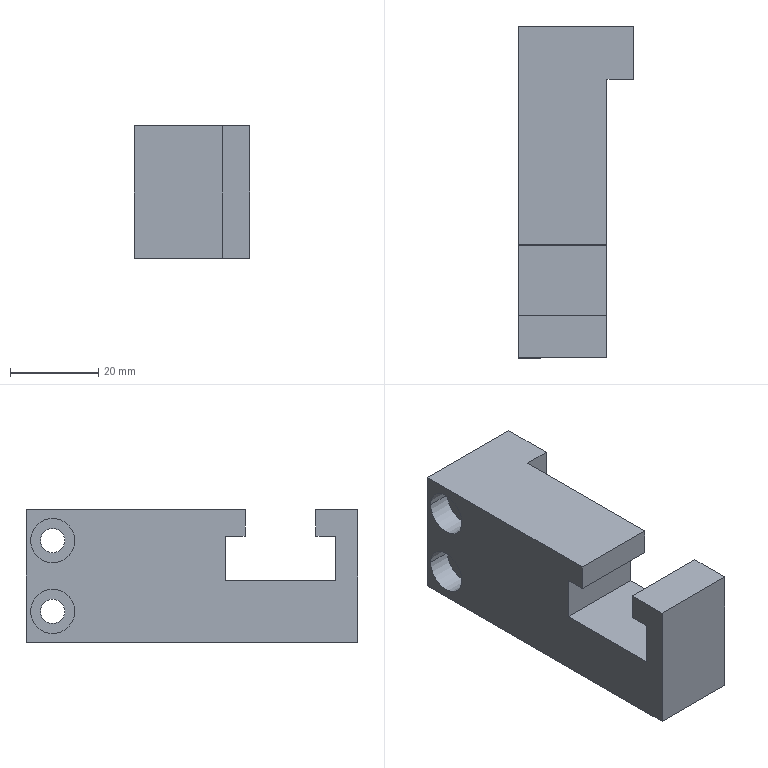Component | SolidWorks | 15-1 | 1 solid | 26 faces | box 26 x 75 x 30 mm | volume 38413 mm3 | plane 18 | cylinder 8 | commonest cylinder face diameters 10 x4 5.5 x4
build123d program:
from build123d import *

# Parameters (mm, degrees)
SKETCH1_W                                       = 30
SKETCH1_H                                       = 75
EXTRUDE1_DEPTH                                  = 10
CUT_EXTRUDE1_DEPTH                              = 46.069
SKETCH3_W                                       = 30
SKETCH3_H                                       = 12
EXTRUDE2_DEPTH                                  = 6
M5_HEX_SOCKET_HEAD_CAP_SCREW_CBORE1_D           = 5.5
M5_HEX_SOCKET_HEAD_CAP_SCREW_CBORE1_CBORE_D     = 10
M5_HEX_SOCKET_HEAD_CAP_SCREW_CBORE1_CBORE_DEPTH = 5.4


with BuildPart() as part:
    # Sketch1 → Extrude1 (new, symmetric)
    with BuildSketch(Plane(origin=(0, 0, 0), x_dir=(1, 0, 0), z_dir=(0, 1, 0))):
        Rectangle(SKETCH1_W, SKETCH1_H)
    extrude(amount=EXTRUDE1_DEPTH, both=True)

    # Sketch2 → Cut-Extrude1 (cut, through all)
    with BuildSketch(Plane.XZ.offset(10)):
        Polygon((15, 28), (9, 28), (9, 32.5), (-1, 32.5), (-1, 7.5), (9, 7.5), (9, 12), (15, 12), align=None)
    extrude(amount=-CUT_EXTRUDE1_DEPTH, mode=Mode.SUBTRACT)

    # Sketch3 → Extrude2 (add)
    with BuildSketch(Plane(origin=(0, -10, 0), x_dir=(1, 0, 0), z_dir=(0, 1, 0))):
        with Locations((0, 31.5)):
            Rectangle(SKETCH3_W, SKETCH3_H)
    extrude(amount=-EXTRUDE2_DEPTH)

    # M5 Hex Socket Head Cap Screw CBORE1 (through all)
    with Locations(Plane(origin=(0, 10, 0), x_dir=(1, 0, 0), z_dir=(0, 1, 0))):
        with Locations((8, 31.5), (-8, 31.5)):
            CounterBoreHole(M5_HEX_SOCKET_HEAD_CAP_SCREW_CBORE1_D / 2, M5_HEX_SOCKET_HEAD_CAP_SCREW_CBORE1_CBORE_D / 2, M5_HEX_SOCKET_HEAD_CAP_SCREW_CBORE1_CBORE_DEPTH)


solid = part.part

# Placed as in the assembly
solid = solid.moved(Location((-103, -9.5, 101.8), (90, 0, 90)))
STEP:
#1=COLOUR_RGB('',0.7922,0.8196,0.9333);
#2=FILL_AREA_STYLE_COLOUR('',#1);
#3=FILL_AREA_STYLE('',(#2));
#4=SURFACE_STYLE_FILL_AREA(#3);
#5=SURFACE_SIDE_STYLE('',(#4));
#6=SURFACE_STYLE_USAGE(.BOTH.,#5);
#7=PRESENTATION_STYLE_ASSIGNMENT((#6));
#8=CARTESIAN_POINT('',(-4.236,1.063,4.323));
#9=VERTEX_POINT('',#8);
#10=CARTESIAN_POINT('',(-4.236,0.6693,4.323));
#11=VERTEX_POINT('',#10);
#12=CARTESIAN_POINT('',(-4.236,0.8661,4.323));
#13=DIRECTION('',(-1.,-0.,0.));
#14=DIRECTION('',(0.,-1.,0.));
#15=AXIS2_PLACEMENT_3D('',#12,#13,#14);
#16=CIRCLE('',#15,0.1969);
#17=EDGE_CURVE('',#9,#11,#16,.T.);
#18=ORIENTED_EDGE('',*,*,#17,.F.);
#19=CARTESIAN_POINT('',(-4.449,1.063,4.323));
#20=VERTEX_POINT('',#19);
#21=CARTESIAN_POINT('',(-4.449,1.063,4.323));
#22=DIRECTION('',(-1.,-0.,0.));
#23=VECTOR('',#22,39.37);
#24=LINE('',#21,#23);
#25=EDGE_CURVE('',#9,#20,#24,.T.);
#26=ORIENTED_EDGE('',*,*,#25,.T.);
#27=CARTESIAN_POINT('',(-4.449,0.6693,4.323));
#28=VERTEX_POINT('',#27);
#29=CARTESIAN_POINT('',(-4.449,0.8661,4.323));
#30=DIRECTION('',(-1.,-0.,0.));
#31=DIRECTION('',(0.,-1.,0.));
#32=AXIS2_PLACEMENT_3D('',#29,#30,#31);
#33=CIRCLE('',#32,0.1969);
#34=EDGE_CURVE('',#20,#28,#33,.T.);
#35=ORIENTED_EDGE('',*,*,#34,.T.);
#36=CARTESIAN_POINT('',(-4.449,0.6693,4.323));
#37=DIRECTION('',(-1.,-0.,0.));
#38=VECTOR('',#37,39.37);
#39=LINE('',#36,#38);
#40=EDGE_CURVE('',#11,#28,#39,.T.);
#41=ORIENTED_EDGE('',*,*,#40,.F.);
#42=EDGE_LOOP('',(#18,#26,#35,#41));
#43=FACE_OUTER_BOUND('',#42,.T.);
#44=CARTESIAN_POINT('',(-4.449,0.8661,4.323));
#45=DIRECTION('',(-1.,-0.,0.));
#46=DIRECTION('',(0.,-1.,0.));
#47=AXIS2_PLACEMENT_3D('',#44,#45,#46);
#48=CYLINDRICAL_SURFACE('',#47,0.1969);
#49=ADVANCED_FACE('',(#43),#48,.F.);
#50=CARTESIAN_POINT('',(-3.425,0.9744,4.323));
#51=VERTEX_POINT('',#50);
#52=CARTESIAN_POINT('',(-3.425,0.7579,4.323));
#53=VERTEX_POINT('',#52);
#54=CARTESIAN_POINT('',(-3.425,0.8661,4.323));
#55=DIRECTION('',(-1.,-0.,0.));
#56=DIRECTION('',(0.,-1.,0.));
#57=AXIS2_PLACEMENT_3D('',#54,#55,#56);
#58=CIRCLE('',#57,0.1083);
#59=EDGE_CURVE('',#51,#53,#58,.T.);
#60=ORIENTED_EDGE('',*,*,#59,.F.);
#61=CARTESIAN_POINT('',(-4.236,0.9744,4.323));
#62=VERTEX_POINT('',#61);
#63=CARTESIAN_POINT('',(-4.449,0.9744,4.323));
#64=DIRECTION('',(-1.,-0.,0.));
#65=VECTOR('',#64,39.37);
#66=LINE('',#63,#65);
#67=EDGE_CURVE('',#51,#62,#66,.T.);
#68=ORIENTED_EDGE('',*,*,#67,.T.);
#69=CARTESIAN_POINT('',(-4.236,0.7579,4.323));
#70=VERTEX_POINT('',#69);
#71=CARTESIAN_POINT('',(-4.236,0.8661,4.323));
#72=DIRECTION('',(-1.,-0.,0.));
#73=DIRECTION('',(0.,-1.,0.));
#74=AXIS2_PLACEMENT_3D('',#71,#72,#73);
#75=CIRCLE('',#74,0.1083);
#76=EDGE_CURVE('',#62,#70,#75,.T.);
#77=ORIENTED_EDGE('',*,*,#76,.T.);
#78=CARTESIAN_POINT('',(-4.449,0.7579,4.323));
#79=DIRECTION('',(-1.,-0.,0.));
#80=VECTOR('',#79,39.37);
#81=LINE('',#78,#80);
#82=EDGE_CURVE('',#53,#70,#81,.T.);
#83=ORIENTED_EDGE('',*,*,#82,.F.);
#84=EDGE_LOOP('',(#60,#68,#77,#83));
#85=FACE_OUTER_BOUND('',#84,.T.);
#86=CARTESIAN_POINT('',(-4.449,0.8661,4.323));
#87=DIRECTION('',(-1.,-0.,0.));
#88=DIRECTION('',(0.,-1.,0.));
#89=AXIS2_PLACEMENT_3D('',#86,#87,#88);
#90=CYLINDRICAL_SURFACE('',#89,0.1083);
#91=ADVANCED_FACE('',(#85),#90,.F.);
#92=CARTESIAN_POINT('',(-4.236,1.063,3.693));
#93=VERTEX_POINT('',#92);
#94=CARTESIAN_POINT('',(-4.236,0.6693,3.693));
#95=VERTEX_POINT('',#94);
#96=CARTESIAN_POINT('',(-4.236,0.8661,3.693));
#97=DIRECTION('',(-1.,-0.,0.));
#98=DIRECTION('',(0.,-1.,0.));
#99=AXIS2_PLACEMENT_3D('',#96,#97,#98);
#100=CIRCLE('',#99,0.1969);
#101=EDGE_CURVE('',#93,#95,#100,.T.);
#102=ORIENTED_EDGE('',*,*,#101,.F.);
#103=CARTESIAN_POINT('',(-4.449,1.063,3.693));
#104=VERTEX_POINT('',#103);
#105=CARTESIAN_POINT('',(-4.449,1.063,3.693));
#106=DIRECTION('',(-1.,-0.,0.));
#107=VECTOR('',#106,39.37);
#108=LINE('',#105,#107);
#109=EDGE_CURVE('',#93,#104,#108,.T.);
#110=ORIENTED_EDGE('',*,*,#109,.T.);
#111=CARTESIAN_POINT('',(-4.449,0.6693,3.693));
#112=VERTEX_POINT('',#111);
#113=CARTESIAN_POINT('',(-4.449,0.8661,3.693));
#114=DIRECTION('',(-1.,-0.,0.));
#115=DIRECTION('',(0.,-1.,0.));
#116=AXIS2_PLACEMENT_3D('',#113,#114,#115);
#117=CIRCLE('',#116,0.1969);
#118=EDGE_CURVE('',#104,#112,#117,.T.);
#119=ORIENTED_EDGE('',*,*,#118,.T.);
#120=CARTESIAN_POINT('',(-4.449,0.6693,3.693));
#121=DIRECTION('',(-1.,-0.,0.));
#122=VECTOR('',#121,39.37);
#123=LINE('',#120,#122);
#124=EDGE_CURVE('',#95,#112,#123,.T.);
#125=ORIENTED_EDGE('',*,*,#124,.F.);
#126=EDGE_LOOP('',(#102,#110,#119,#125));
#127=FACE_OUTER_BOUND('',#126,.T.);
#128=CARTESIAN_POINT('',(-4.449,0.8661,3.693));
#129=DIRECTION('',(-1.,-0.,0.));
#130=DIRECTION('',(0.,-1.,0.));
#131=AXIS2_PLACEMENT_3D('',#128,#129,#130);
#132=CYLINDRICAL_SURFACE('',#131,0.1969);
#133=ADVANCED_FACE('',(#127),#132,.F.);
#134=CARTESIAN_POINT('',(-3.425,0.9744,3.693));
#135=VERTEX_POINT('',#134);
#136=CARTESIAN_POINT('',(-3.425,0.7579,3.693));
#137=VERTEX_POINT('',#136);
#138=CARTESIAN_POINT('',(-3.425,0.8661,3.693));
#139=DIRECTION('',(-1.,-0.,0.));
#140=DIRECTION('',(0.,-1.,0.));
#141=AXIS2_PLACEMENT_3D('',#138,#139,#140);
#142=CIRCLE('',#141,0.1083);
#143=EDGE_CURVE('',#135,#137,#142,.T.);
#144=ORIENTED_EDGE('',*,*,#143,.F.);
#145=CARTESIAN_POINT('',(-4.236,0.9744,3.693));
#146=VERTEX_POINT('',#145);
#147=CARTESIAN_POINT('',(-4.449,0.9744,3.693));
#148=DIRECTION('',(-1.,-0.,0.));
#149=VECTOR('',#148,39.37);
#150=LINE('',#147,#149);
#151=EDGE_CURVE('',#135,#146,#150,.T.);
#152=ORIENTED_EDGE('',*,*,#151,.T.);
#153=CARTESIAN_POINT('',(-4.236,0.7579,3.693));
#154=VERTEX_POINT('',#153);
#155=CARTESIAN_POINT('',(-4.236,0.8661,3.693));
#156=DIRECTION('',(-1.,-0.,0.));
#157=DIRECTION('',(0.,-1.,0.));
#158=AXIS2_PLACEMENT_3D('',#155,#156,#157);
#159=CIRCLE('',#158,0.1083);
#160=EDGE_CURVE('',#146,#154,#159,.T.);
#161=ORIENTED_EDGE('',*,*,#160,.T.);
#162=CARTESIAN_POINT('',(-4.449,0.7579,3.693));
#163=DIRECTION('',(-1.,-0.,0.));
#164=VECTOR('',#163,39.37);
#165=LINE('',#162,#164);
#166=EDGE_CURVE('',#137,#154,#165,.T.);
#167=ORIENTED_EDGE('',*,*,#166,.F.);
#168=EDGE_LOOP('',(#144,#152,#161,#167));
#169=FACE_OUTER_BOUND('',#168,.T.);
#170=CARTESIAN_POINT('',(-4.449,0.8661,3.693));
#171=DIRECTION('',(-1.,-0.,0.));
#172=DIRECTION('',(0.,-1.,0.));
#173=AXIS2_PLACEMENT_3D('',#170,#171,#172);
#174=CYLINDRICAL_SURFACE('',#173,0.1083);
#175=ADVANCED_FACE('',(#169),#174,.F.);
#176=CARTESIAN_POINT('',(-4.449,-0.8465,4.598));
#177=VERTEX_POINT('',#176);
#178=CARTESIAN_POINT('',(-4.449,1.102,4.598));
#179=VERTEX_POINT('',#178);
#180=CARTESIAN_POINT('',(-4.449,1.102,4.598));
#181=DIRECTION('',(-0.,1.,-0.));
#182=VECTOR('',#181,39.37);
#183=LINE('',#180,#182);
#184=EDGE_CURVE('',#177,#179,#183,.T.);
#185=ORIENTED_EDGE('',*,*,#184,.F.);
#186=CARTESIAN_POINT('',(-3.661,-0.8465,4.598));
#187=VERTEX_POINT('',#186);
#188=CARTESIAN_POINT('',(-4.449,-0.8465,4.598));
#189=DIRECTION('',(1.,0.,-0.));
#190=VECTOR('',#189,39.37);
#191=LINE('',#188,#190);
#192=EDGE_CURVE('',#177,#187,#191,.T.);
#193=ORIENTED_EDGE('',*,*,#192,.T.);
#194=CARTESIAN_POINT('',(-3.661,0.6299,4.598));
#195=VERTEX_POINT('',#194);
#196=CARTESIAN_POINT('',(-3.661,1.102,4.598));
#197=DIRECTION('',(-0.,1.,-0.));
#198=VECTOR('',#197,39.37);
#199=LINE('',#196,#198);
#200=EDGE_CURVE('',#187,#195,#199,.T.);
#201=ORIENTED_EDGE('',*,*,#200,.T.);
#202=CARTESIAN_POINT('',(-3.425,0.6299,4.598));
#203=VERTEX_POINT('',#202);
#204=CARTESIAN_POINT('',(-3.425,0.6299,4.598));
#205=DIRECTION('',(-1.,-0.,0.));
#206=VECTOR('',#205,39.37);
#207=LINE('',#204,#206);
#208=EDGE_CURVE('',#203,#195,#207,.T.);
#209=ORIENTED_EDGE('',*,*,#208,.F.);
#210=CARTESIAN_POINT('',(-3.425,1.102,4.598));
#211=VERTEX_POINT('',#210);
#212=CARTESIAN_POINT('',(-3.425,1.102,4.598));
#213=DIRECTION('',(-0.,1.,-0.));
#214=VECTOR('',#213,39.37);
#215=LINE('',#212,#214);
#216=EDGE_CURVE('',#203,#211,#215,.T.);
#217=ORIENTED_EDGE('',*,*,#216,.T.);
#218=CARTESIAN_POINT('',(-4.449,1.102,4.598));
#219=DIRECTION('',(1.,0.,-0.));
#220=VECTOR('',#219,39.37);
#221=LINE('',#218,#220);
#222=EDGE_CURVE('',#179,#211,#221,.T.);
#223=ORIENTED_EDGE('',*,*,#222,.F.);
#224=EDGE_LOOP('',(#185,#193,#201,#209,#217,#223));
#225=FACE_OUTER_BOUND('',#224,.T.);
#226=CARTESIAN_POINT('',(-4.449,1.102,4.598));
#227=DIRECTION('',(-0.,-0.,-1.));
#228=DIRECTION('',(0.,-1.,0.));
#229=AXIS2_PLACEMENT_3D('',#226,#227,#228);
#230=PLANE('',#229);
#231=ADVANCED_FACE('',(#225),#230,.F.);
#232=CARTESIAN_POINT('',(-4.449,1.102,3.417));
#233=VERTEX_POINT('',#232);
#234=CARTESIAN_POINT('',(-3.425,1.102,3.417));
#235=VERTEX_POINT('',#234);
#236=CARTESIAN_POINT('',(-4.449,1.102,3.417));
#237=DIRECTION('',(1.,0.,-0.));
#238=VECTOR('',#237,39.37);
#239=LINE('',#236,#238);
#240=EDGE_CURVE('',#233,#235,#239,.T.);
#241=ORIENTED_EDGE('',*,*,#240,.T.);
#242=CARTESIAN_POINT('',(-3.425,0.6299,3.417));
#243=VERTEX_POINT('',#242);
#244=CARTESIAN_POINT('',(-3.425,1.102,3.417));
#245=DIRECTION('',(0.,-1.,0.));
#246=VECTOR('',#245,39.37);
#247=LINE('',#244,#246);
#248=EDGE_CURVE('',#235,#243,#247,.T.);
#249=ORIENTED_EDGE('',*,*,#248,.T.);
#250=CARTESIAN_POINT('',(-3.661,0.6299,3.417));
#251=VERTEX_POINT('',#250);
#252=CARTESIAN_POINT('',(-3.425,0.6299,3.417));
#253=DIRECTION('',(-1.,-0.,0.));
#254=VECTOR('',#253,39.37);
#255=LINE('',#252,#254);
#256=EDGE_CURVE('',#243,#251,#255,.T.);
#257=ORIENTED_EDGE('',*,*,#256,.T.);
#258=CARTESIAN_POINT('',(-3.661,-1.85,3.417));
#259=VERTEX_POINT('',#258);
#260=CARTESIAN_POINT('',(-3.661,1.102,3.417));
#261=DIRECTION('',(0.,-1.,0.));
#262=VECTOR('',#261,39.37);
#263=LINE('',#260,#262);
#264=EDGE_CURVE('',#251,#259,#263,.T.);
#265=ORIENTED_EDGE('',*,*,#264,.T.);
#266=CARTESIAN_POINT('',(-4.449,-1.85,3.417));
#267=VERTEX_POINT('',#266);
#268=CARTESIAN_POINT('',(-4.449,-1.85,3.417));
#269=DIRECTION('',(1.,0.,-0.));
#270=VECTOR('',#269,39.37);
#271=LINE('',#268,#270);
#272=EDGE_CURVE('',#267,#259,#271,.T.);
#273=ORIENTED_EDGE('',*,*,#272,.F.);
#274=CARTESIAN_POINT('',(-4.449,1.102,3.417));
#275=DIRECTION('',(0.,-1.,0.));
#276=VECTOR('',#275,39.37);
#277=LINE('',#274,#276);
#278=EDGE_CURVE('',#233,#267,#277,.T.);
#279=ORIENTED_EDGE('',*,*,#278,.F.);
#280=EDGE_LOOP('',(#241,#249,#257,#265,#273,#279));
#281=FACE_OUTER_BOUND('',#280,.T.);
#282=CARTESIAN_POINT('',(-4.449,1.102,3.417));
#283=DIRECTION('',(0.,0.,1.));
#284=DIRECTION('',(-0.,1.,-0.));
#285=AXIS2_PLACEMENT_3D('',#282,#283,#284);
#286=PLANE('',#285);
#287=ADVANCED_FACE('',(#281),#286,.F.);
#288=CARTESIAN_POINT('',(-3.661,-1.85,4.598));
#289=VERTEX_POINT('',#288);
#290=CARTESIAN_POINT('',(-3.661,-1.85,3.417));
#291=DIRECTION('',(0.,0.,1.));
#292=VECTOR('',#291,39.37);
#293=LINE('',#290,#292);
#294=EDGE_CURVE('',#259,#289,#293,.T.);
#295=ORIENTED_EDGE('',*,*,#294,.T.);
#296=CARTESIAN_POINT('',(-4.449,-1.85,4.598));
#297=VERTEX_POINT('',#296);
#298=CARTESIAN_POINT('',(-4.449,-1.85,4.598));
#299=DIRECTION('',(1.,0.,-0.));
#300=VECTOR('',#299,39.37);
#301=LINE('',#298,#300);
#302=EDGE_CURVE('',#297,#289,#301,.T.);
#303=ORIENTED_EDGE('',*,*,#302,.F.);
#304=CARTESIAN_POINT('',(-4.449,-1.85,3.417));
#305=DIRECTION('',(0.,0.,1.));
#306=VECTOR('',#305,39.37);
#307=LINE('',#304,#306);
#308=EDGE_CURVE('',#267,#297,#307,.T.);
#309=ORIENTED_EDGE('',*,*,#308,.F.);
#310=ORIENTED_EDGE('',*,*,#272,.T.);
#311=EDGE_LOOP('',(#295,#303,#309,#310));
#312=FACE_OUTER_BOUND('',#311,.T.);
#313=CARTESIAN_POINT('',(-4.449,-1.85,3.417));
#314=DIRECTION('',(-0.,1.,-0.));
#315=DIRECTION('',(-0.,-0.,-1.));
#316=AXIS2_PLACEMENT_3D('',#313,#314,#315);
#317=PLANE('',#316);
#318=ADVANCED_FACE('',(#312),#317,.F.);
#319=CARTESIAN_POINT('',(-3.661,-1.476,4.598));
#320=VERTEX_POINT('',#319);
#321=CARTESIAN_POINT('',(-3.661,1.102,4.598));
#322=DIRECTION('',(-0.,1.,-0.));
#323=VECTOR('',#322,39.37);
#324=LINE('',#321,#323);
#325=EDGE_CURVE('',#289,#320,#324,.T.);
#326=ORIENTED_EDGE('',*,*,#325,.T.);
#327=CARTESIAN_POINT('',(-4.449,-1.476,4.598));
#328=VERTEX_POINT('',#327);
#329=CARTESIAN_POINT('',(-4.449,-1.476,4.598));
#330=DIRECTION('',(1.,0.,-0.));
#331=VECTOR('',#330,39.37);
#332=LINE('',#329,#331);
#333=EDGE_CURVE('',#328,#320,#332,.T.);
#334=ORIENTED_EDGE('',*,*,#333,.F.);
#335=CARTESIAN_POINT('',(-4.449,1.102,4.598));
#336=DIRECTION('',(-0.,1.,-0.));
#337=VECTOR('',#336,39.37);
#338=LINE('',#335,#337);
#339=EDGE_CURVE('',#297,#328,#338,.T.);
#340=ORIENTED_EDGE('',*,*,#339,.F.);
#341=ORIENTED_EDGE('',*,*,#302,.T.);
#342=EDGE_LOOP('',(#326,#334,#340,#341));
#343=FACE_OUTER_BOUND('',#342,.T.);
#344=CARTESIAN_POINT('',(-4.449,1.102,4.598));
#345=DIRECTION('',(-0.,-0.,-1.));
#346=DIRECTION('',(0.,-1.,0.));
#347=AXIS2_PLACEMENT_3D('',#344,#345,#346);
#348=PLANE('',#347);
#349=ADVANCED_FACE('',(#343),#348,.F.);
#350=ORIENTED_EDGE('',*,*,#222,.T.);
#351=CARTESIAN_POINT('',(-3.425,1.102,3.417));
#352=DIRECTION('',(-0.,-0.,-1.));
#353=VECTOR('',#352,39.37);
#354=LINE('',#351,#353);
#355=EDGE_CURVE('',#211,#235,#354,.T.);
#356=ORIENTED_EDGE('',*,*,#355,.T.);
#357=ORIENTED_EDGE('',*,*,#240,.F.);
#358=CARTESIAN_POINT('',(-4.449,1.102,3.417));
#359=DIRECTION('',(-0.,-0.,-1.));
#360=VECTOR('',#359,39.37);
#361=LINE('',#358,#360);
#362=EDGE_CURVE('',#179,#233,#361,.T.);
#363=ORIENTED_EDGE('',*,*,#362,.F.);
#364=EDGE_LOOP('',(#350,#356,#357,#363));
#365=FACE_OUTER_BOUND('',#364,.T.);
#366=CARTESIAN_POINT('',(-4.449,1.102,3.417));
#367=DIRECTION('',(0.,-1.,0.));
#368=DIRECTION('',(0.,0.,1.));
#369=AXIS2_PLACEMENT_3D('',#366,#367,#368);
#370=PLANE('',#369);
#371=ADVANCED_FACE('',(#365),#370,.F.);
#372=CARTESIAN_POINT('',(-4.449,0.8661,4.323));
#373=DIRECTION('',(-1.,-0.,0.));
#374=DIRECTION('',(0.,-1.,0.));
#375=AXIS2_PLACEMENT_3D('',#372,#373,#374);
#376=CIRCLE('',#375,0.1969);
#377=EDGE_CURVE('',#28,#20,#376,.T.);
#378=ORIENTED_EDGE('',*,*,#377,.F.);
#379=ORIENTED_EDGE('',*,*,#34,.F.);
#380=EDGE_LOOP('',(#378,#379));
#381=FACE_BOUND('',#380,.T.);
#382=CARTESIAN_POINT('',(-4.449,0.8661,3.693));
#383=DIRECTION('',(-1.,-0.,0.));
#384=DIRECTION('',(0.,-1.,0.));
#385=AXIS2_PLACEMENT_3D('',#382,#383,#384);
#386=CIRCLE('',#385,0.1969);
#387=EDGE_CURVE('',#112,#104,#386,.T.);
#388=ORIENTED_EDGE('',*,*,#387,.F.);
#389=ORIENTED_EDGE('',*,*,#118,.F.);
#390=EDGE_LOOP('',(#388,#389));
#391=FACE_BOUND('',#390,.T.);
#392=CARTESIAN_POINT('',(-4.449,-0.8465,4.362));
#393=VERTEX_POINT('',#392);
#394=CARTESIAN_POINT('',(-4.449,-0.8465,4.362));
#395=DIRECTION('',(0.,0.,1.));
#396=VECTOR('',#395,39.37);
#397=LINE('',#394,#396);
#398=EDGE_CURVE('',#393,#177,#397,.T.);
#399=ORIENTED_EDGE('',*,*,#398,.T.);
#400=ORIENTED_EDGE('',*,*,#184,.T.);
#401=ORIENTED_EDGE('',*,*,#362,.T.);
#402=ORIENTED_EDGE('',*,*,#278,.T.);
#403=ORIENTED_EDGE('',*,*,#308,.T.);
#404=ORIENTED_EDGE('',*,*,#339,.T.);
#405=CARTESIAN_POINT('',(-4.449,-1.476,4.362));
#406=VERTEX_POINT('',#405);
#407=CARTESIAN_POINT('',(-4.449,-1.476,4.598));
#408=DIRECTION('',(-0.,-0.,-1.));
#409=VECTOR('',#408,39.37);
#410=LINE('',#407,#409);
#411=EDGE_CURVE('',#328,#406,#410,.T.);
#412=ORIENTED_EDGE('',*,*,#411,.T.);
#413=CARTESIAN_POINT('',(-4.449,-1.654,4.362));
#414=VERTEX_POINT('',#413);
#415=CARTESIAN_POINT('',(-4.449,-1.476,4.362));
#416=DIRECTION('',(0.,-1.,0.));
#417=VECTOR('',#416,39.37);
#418=LINE('',#415,#417);
#419=EDGE_CURVE('',#406,#414,#418,.T.);
#420=ORIENTED_EDGE('',*,*,#419,.T.);
#421=CARTESIAN_POINT('',(-4.449,-1.654,3.969));
#422=VERTEX_POINT('',#421);
#423=CARTESIAN_POINT('',(-4.449,-1.654,4.362));
#424=DIRECTION('',(-0.,-0.,-1.));
#425=VECTOR('',#424,39.37);
#426=LINE('',#423,#425);
#427=EDGE_CURVE('',#414,#422,#426,.T.);
#428=ORIENTED_EDGE('',*,*,#427,.T.);
#429=CARTESIAN_POINT('',(-4.449,-0.6693,3.969));
#430=VERTEX_POINT('',#429);
#431=CARTESIAN_POINT('',(-4.449,-1.654,3.969));
#432=DIRECTION('',(-0.,1.,-0.));
#433=VECTOR('',#432,39.37);
#434=LINE('',#431,#433);
#435=EDGE_CURVE('',#422,#430,#434,.T.);
#436=ORIENTED_EDGE('',*,*,#435,.T.);
#437=CARTESIAN_POINT('',(-4.449,-0.6693,4.362));
#438=VERTEX_POINT('',#437);
#439=CARTESIAN_POINT('',(-4.449,-0.6693,3.969));
#440=DIRECTION('',(0.,0.,1.));
#441=VECTOR('',#440,39.37);
#442=LINE('',#439,#441);
#443=EDGE_CURVE('',#430,#438,#442,.T.);
#444=ORIENTED_EDGE('',*,*,#443,.T.);
#445=CARTESIAN_POINT('',(-4.449,-0.6693,4.362));
#446=DIRECTION('',(0.,-1.,0.));
#447=VECTOR('',#446,39.37);
#448=LINE('',#445,#447);
#449=EDGE_CURVE('',#438,#393,#448,.T.);
#450=ORIENTED_EDGE('',*,*,#449,.T.);
#451=EDGE_LOOP('',(#399,#400,#401,#402,#403,#404,#412,#420,#428,#436,#444,#450));
#452=FACE_OUTER_BOUND('',#451,.T.);
#453=CARTESIAN_POINT('',(-4.449,-0.374,4.008));
#454=DIRECTION('',(-1.,-0.,0.));
#455=DIRECTION('',(0.,-1.,0.));
#456=AXIS2_PLACEMENT_3D('',#453,#454,#455);
#457=PLANE('',#456);
#458=ADVANCED_FACE('',(#381,#391,#452),#457,.T.);
#459=ORIENTED_EDGE('',*,*,#264,.F.);
#460=CARTESIAN_POINT('',(-3.661,0.6299,3.417));
#461=DIRECTION('',(0.,0.,1.));
#462=VECTOR('',#461,39.37);
#463=LINE('',#460,#462);
#464=EDGE_CURVE('',#251,#195,#463,.T.);
#465=ORIENTED_EDGE('',*,*,#464,.T.);
#466=ORIENTED_EDGE('',*,*,#200,.F.);
#467=CARTESIAN_POINT('',(-3.661,-0.8465,4.362));
#468=VERTEX_POINT('',#467);
#469=CARTESIAN_POINT('',(-3.661,-0.8465,4.362));
#470=DIRECTION('',(0.,0.,1.));
#471=VECTOR('',#470,39.37);
#472=LINE('',#469,#471);
#473=EDGE_CURVE('',#468,#187,#472,.T.);
#474=ORIENTED_EDGE('',*,*,#473,.F.);
#475=CARTESIAN_POINT('',(-3.661,-0.6693,4.362));
#476=VERTEX_POINT('',#475);
#477=CARTESIAN_POINT('',(-3.661,-0.6693,4.362));
#478=DIRECTION('',(0.,-1.,0.));
#479=VECTOR('',#478,39.37);
#480=LINE('',#477,#479);
#481=EDGE_CURVE('',#476,#468,#480,.T.);
#482=ORIENTED_EDGE('',*,*,#481,.F.);
#483=CARTESIAN_POINT('',(-3.661,-0.6693,3.969));
#484=VERTEX_POINT('',#483);
#485=CARTESIAN_POINT('',(-3.661,-0.6693,3.969));
#486=DIRECTION('',(0.,0.,1.));
#487=VECTOR('',#486,39.37);
#488=LINE('',#485,#487);
#489=EDGE_CURVE('',#484,#476,#488,.T.);
#490=ORIENTED_EDGE('',*,*,#489,.F.);
#491=CARTESIAN_POINT('',(-3.661,-1.654,3.969));
#492=VERTEX_POINT('',#491);
#493=CARTESIAN_POINT('',(-3.661,-1.654,3.969));
#494=DIRECTION('',(-0.,1.,-0.));
#495=VECTOR('',#494,39.37);
#496=LINE('',#493,#495);
#497=EDGE_CURVE('',#492,#484,#496,.T.);
#498=ORIENTED_EDGE('',*,*,#497,.F.);
#499=CARTESIAN_POINT('',(-3.661,-1.654,4.362));
#500=VERTEX_POINT('',#499);
#501=CARTESIAN_POINT('',(-3.661,-1.654,4.362));
#502=DIRECTION('',(-0.,-0.,-1.));
#503=VECTOR('',#502,39.37);
#504=LINE('',#501,#503);
#505=EDGE_CURVE('',#500,#492,#504,.T.);
#506=ORIENTED_EDGE('',*,*,#505,.F.);
#507=CARTESIAN_POINT('',(-3.661,-1.476,4.362));
#508=VERTEX_POINT('',#507);
#509=CARTESIAN_POINT('',(-3.661,-1.476,4.362));
#510=DIRECTION('',(0.,-1.,0.));
#511=VECTOR('',#510,39.37);
#512=LINE('',#509,#511);
#513=EDGE_CURVE('',#508,#500,#512,.T.);
#514=ORIENTED_EDGE('',*,*,#513,.F.);
#515=CARTESIAN_POINT('',(-3.661,-1.476,4.598));
#516=DIRECTION('',(-0.,-0.,-1.));
#517=VECTOR('',#516,39.37);
#518=LINE('',#515,#517);
#519=EDGE_CURVE('',#320,#508,#518,.T.);
#520=ORIENTED_EDGE('',*,*,#519,.F.);
#521=ORIENTED_EDGE('',*,*,#325,.F.);
#522=ORIENTED_EDGE('',*,*,#294,.F.);
#523=EDGE_LOOP('',(#459,#465,#466,#474,#482,#490,#498,#506,#514,#520,#521,#522));
#524=FACE_OUTER_BOUND('',#523,.T.);
#525=CARTESIAN_POINT('',(-3.661,-0.374,4.008));
#526=DIRECTION('',(-1.,-0.,0.));
#527=DIRECTION('',(0.,-1.,0.));
#528=AXIS2_PLACEMENT_3D('',#525,#526,#527);
#529=PLANE('',#528);
#530=ADVANCED_FACE('',(#524),#529,.F.);
#531=ORIENTED_EDGE('',*,*,#473,.T.);
#532=ORIENTED_EDGE('',*,*,#192,.F.);
#533=ORIENTED_EDGE('',*,*,#398,.F.);
#534=CARTESIAN_POINT('',(-4.449,-0.8465,4.362));
#535=DIRECTION('',(1.,0.,-0.));
#536=VECTOR('',#535,39.37);
#537=LINE('',#534,#536);
#538=EDGE_CURVE('',#393,#468,#537,.T.);
#539=ORIENTED_EDGE('',*,*,#538,.T.);
#540=EDGE_LOOP('',(#531,#532,#533,#539));
#541=FACE_OUTER_BOUND('',#540,.T.);
#542=CARTESIAN_POINT('',(-4.449,-0.8465,4.362));
#543=DIRECTION('',(-0.,1.,-0.));
#544=DIRECTION('',(-0.,-0.,-1.));
#545=AXIS2_PLACEMENT_3D('',#542,#543,#544);
#546=PLANE('',#545);
#547=ADVANCED_FACE('',(#541),#546,.F.);
#548=ORIENTED_EDGE('',*,*,#481,.T.);
#549=ORIENTED_EDGE('',*,*,#538,.F.);
#550=ORIENTED_EDGE('',*,*,#449,.F.);
#551=CARTESIAN_POINT('',(-4.449,-0.6693,4.362));
#552=DIRECTION('',(1.,0.,-0.));
#553=VECTOR('',#552,39.37);
#554=LINE('',#551,#553);
#555=EDGE_CURVE('',#438,#476,#554,.T.);
#556=ORIENTED_EDGE('',*,*,#555,.T.);
#557=EDGE_LOOP('',(#548,#549,#550,#556));
#558=FACE_OUTER_BOUND('',#557,.T.);
#559=CARTESIAN_POINT('',(-4.449,-0.6693,4.362));
#560=DIRECTION('',(0.,0.,1.));
#561=DIRECTION('',(-0.,1.,-0.));
#562=AXIS2_PLACEMENT_3D('',#559,#560,#561);
#563=PLANE('',#562);
#564=ADVANCED_FACE('',(#558),#563,.F.);
#565=ORIENTED_EDGE('',*,*,#489,.T.);
#566=ORIENTED_EDGE('',*,*,#555,.F.);
#567=ORIENTED_EDGE('',*,*,#443,.F.);
#568=CARTESIAN_POINT('',(-4.449,-0.6693,3.969));
#569=DIRECTION('',(1.,0.,-0.));
#570=VECTOR('',#569,39.37);
#571=LINE('',#568,#570);
#572=EDGE_CURVE('',#430,#484,#571,.T.);
#573=ORIENTED_EDGE('',*,*,#572,.T.);
#574=EDGE_LOOP('',(#565,#566,#567,#573));
#575=FACE_OUTER_BOUND('',#574,.T.);
#576=CARTESIAN_POINT('',(-4.449,-0.6693,3.969));
#577=DIRECTION('',(-0.,1.,-0.));
#578=DIRECTION('',(-0.,-0.,-1.));
#579=AXIS2_PLACEMENT_3D('',#576,#577,#578);
#580=PLANE('',#579);
#581=ADVANCED_FACE('',(#575),#580,.F.);
#582=ORIENTED_EDGE('',*,*,#497,.T.);
#583=ORIENTED_EDGE('',*,*,#572,.F.);
#584=ORIENTED_EDGE('',*,*,#435,.F.);
#585=CARTESIAN_POINT('',(-4.449,-1.654,3.969));
#586=DIRECTION('',(1.,0.,-0.));
#587=VECTOR('',#586,39.37);
#588=LINE('',#585,#587);
#589=EDGE_CURVE('',#422,#492,#588,.T.);
#590=ORIENTED_EDGE('',*,*,#589,.T.);
#591=EDGE_LOOP('',(#582,#583,#584,#590));
#592=FACE_OUTER_BOUND('',#591,.T.);
#593=CARTESIAN_POINT('',(-4.449,-1.654,3.969));
#594=DIRECTION('',(-0.,-0.,-1.));
#595=DIRECTION('',(0.,-1.,0.));
#596=AXIS2_PLACEMENT_3D('',#593,#594,#595);
#597=PLANE('',#596);
#598=ADVANCED_FACE('',(#592),#597,.F.);
#599=ORIENTED_EDGE('',*,*,#505,.T.);
#600=ORIENTED_EDGE('',*,*,#589,.F.);
#601=ORIENTED_EDGE('',*,*,#427,.F.);
#602=CARTESIAN_POINT('',(-4.449,-1.654,4.362));
#603=DIRECTION('',(1.,0.,-0.));
#604=VECTOR('',#603,39.37);
#605=LINE('',#602,#604);
#606=EDGE_CURVE('',#414,#500,#605,.T.);
#607=ORIENTED_EDGE('',*,*,#606,.T.);
#608=EDGE_LOOP('',(#599,#600,#601,#607));
#609=FACE_OUTER_BOUND('',#608,.T.);
#610=CARTESIAN_POINT('',(-4.449,-1.654,4.362));
#611=DIRECTION('',(0.,-1.,0.));
#612=DIRECTION('',(0.,0.,1.));
#613=AXIS2_PLACEMENT_3D('',#610,#611,#612);
#614=PLANE('',#613);
#615=ADVANCED_FACE('',(#609),#614,.F.);
#616=ORIENTED_EDGE('',*,*,#513,.T.);
#617=ORIENTED_EDGE('',*,*,#606,.F.);
#618=ORIENTED_EDGE('',*,*,#419,.F.);
#619=CARTESIAN_POINT('',(-4.449,-1.476,4.362));
#620=DIRECTION('',(1.,0.,-0.));
#621=VECTOR('',#620,39.37);
#622=LINE('',#619,#621);
#623=EDGE_CURVE('',#406,#508,#622,.T.);
#624=ORIENTED_EDGE('',*,*,#623,.T.);
#625=EDGE_LOOP('',(#616,#617,#618,#624));
#626=FACE_OUTER_BOUND('',#625,.T.);
#627=CARTESIAN_POINT('',(-4.449,-1.476,4.362));
#628=DIRECTION('',(0.,0.,1.));
#629=DIRECTION('',(-0.,1.,-0.));
#630=AXIS2_PLACEMENT_3D('',#627,#628,#629);
#631=PLANE('',#630);
#632=ADVANCED_FACE('',(#626),#631,.F.);
#633=ORIENTED_EDGE('',*,*,#519,.T.);
#634=ORIENTED_EDGE('',*,*,#623,.F.);
#635=ORIENTED_EDGE('',*,*,#411,.F.);
#636=ORIENTED_EDGE('',*,*,#333,.T.);
#637=EDGE_LOOP('',(#633,#634,#635,#636));
#638=FACE_OUTER_BOUND('',#637,.T.);
#639=CARTESIAN_POINT('',(-4.449,-1.476,4.598));
#640=DIRECTION('',(0.,-1.,0.));
#641=DIRECTION('',(0.,0.,1.));
#642=AXIS2_PLACEMENT_3D('',#639,#640,#641);
#643=PLANE('',#642);
#644=ADVANCED_FACE('',(#638),#643,.F.);
#645=ORIENTED_EDGE('',*,*,#464,.F.);
#646=ORIENTED_EDGE('',*,*,#256,.F.);
#647=CARTESIAN_POINT('',(-3.425,0.6299,3.417));
#648=DIRECTION('',(0.,0.,1.));
#649=VECTOR('',#648,39.37);
#650=LINE('',#647,#649);
#651=EDGE_CURVE('',#243,#203,#650,.T.);
#652=ORIENTED_EDGE('',*,*,#651,.T.);
#653=ORIENTED_EDGE('',*,*,#208,.T.);
#654=EDGE_LOOP('',(#645,#646,#652,#653));
#655=FACE_OUTER_BOUND('',#654,.T.);
#656=CARTESIAN_POINT('',(-3.425,0.6299,3.417));
#657=DIRECTION('',(0.,-1.,0.));
#658=DIRECTION('',(0.,0.,1.));
#659=AXIS2_PLACEMENT_3D('',#656,#657,#658);
#660=PLANE('',#659);
#661=ADVANCED_FACE('',(#655),#660,.T.);
#662=CARTESIAN_POINT('',(-3.425,0.8661,4.323));
#663=DIRECTION('',(-1.,-0.,0.));
#664=DIRECTION('',(0.,-1.,0.));
#665=AXIS2_PLACEMENT_3D('',#662,#663,#664);
#666=CIRCLE('',#665,0.1083);
#667=EDGE_CURVE('',#53,#51,#666,.T.);
#668=ORIENTED_EDGE('',*,*,#667,.T.);
#669=ORIENTED_EDGE('',*,*,#59,.T.);
#670=EDGE_LOOP('',(#668,#669));
#671=FACE_BOUND('',#670,.T.);
#672=CARTESIAN_POINT('',(-3.425,0.8661,3.693));
#673=DIRECTION('',(-1.,-0.,0.));
#674=DIRECTION('',(0.,-1.,0.));
#675=AXIS2_PLACEMENT_3D('',#672,#673,#674);
#676=CIRCLE('',#675,0.1083);
#677=EDGE_CURVE('',#137,#135,#676,.T.);
#678=ORIENTED_EDGE('',*,*,#677,.T.);
#679=ORIENTED_EDGE('',*,*,#143,.T.);
#680=EDGE_LOOP('',(#678,#679));
#681=FACE_BOUND('',#680,.T.);
#682=ORIENTED_EDGE('',*,*,#248,.F.);
#683=ORIENTED_EDGE('',*,*,#355,.F.);
#684=ORIENTED_EDGE('',*,*,#216,.F.);
#685=ORIENTED_EDGE('',*,*,#651,.F.);
#686=EDGE_LOOP('',(#682,#683,#684,#685));
#687=FACE_OUTER_BOUND('',#686,.T.);
#688=CARTESIAN_POINT('',(-3.425,-0.374,4.008));
#689=DIRECTION('',(-1.,-0.,0.));
#690=DIRECTION('',(0.,-1.,0.));
#691=AXIS2_PLACEMENT_3D('',#688,#689,#690);
#692=PLANE('',#691);
#693=ADVANCED_FACE('',(#671,#681,#687),#692,.F.);
#694=ORIENTED_EDGE('',*,*,#151,.F.);
#695=ORIENTED_EDGE('',*,*,#677,.F.);
#696=ORIENTED_EDGE('',*,*,#166,.T.);
#697=CARTESIAN_POINT('',(-4.236,0.8661,3.693));
#698=DIRECTION('',(-1.,-0.,0.));
#699=DIRECTION('',(0.,-1.,0.));
#700=AXIS2_PLACEMENT_3D('',#697,#698,#699);
#701=CIRCLE('',#700,0.1083);
#702=EDGE_CURVE('',#154,#146,#701,.T.);
#703=ORIENTED_EDGE('',*,*,#702,.T.);
#704=EDGE_LOOP('',(#694,#695,#696,#703));
#705=FACE_OUTER_BOUND('',#704,.T.);
#706=CARTESIAN_POINT('',(-4.449,0.8661,3.693));
#707=DIRECTION('',(-1.,-0.,0.));
#708=DIRECTION('',(0.,-1.,0.));
#709=AXIS2_PLACEMENT_3D('',#706,#707,#708);
#710=CYLINDRICAL_SURFACE('',#709,0.1083);
#711=ADVANCED_FACE('',(#705),#710,.F.);
#712=ORIENTED_EDGE('',*,*,#702,.F.);
#713=ORIENTED_EDGE('',*,*,#160,.F.);
#714=EDGE_LOOP('',(#712,#713));
#715=FACE_BOUND('',#714,.T.);
#716=CARTESIAN_POINT('',(-4.236,0.8661,3.693));
#717=DIRECTION('',(-1.,-0.,0.));
#718=DIRECTION('',(0.,-1.,0.));
#719=AXIS2_PLACEMENT_3D('',#716,#717,#718);
#720=CIRCLE('',#719,0.1969);
#721=EDGE_CURVE('',#95,#93,#720,.T.);
#722=ORIENTED_EDGE('',*,*,#721,.T.);
#723=ORIENTED_EDGE('',*,*,#101,.T.);
#724=EDGE_LOOP('',(#722,#723));
#725=FACE_OUTER_BOUND('',#724,.T.);
#726=CARTESIAN_POINT('',(-4.236,0.8661,3.801));
#727=DIRECTION('',(1.,0.,-0.));
#728=DIRECTION('',(-0.,1.,-0.));
#729=AXIS2_PLACEMENT_3D('',#726,#727,#728);
#730=PLANE('',#729);
#731=ADVANCED_FACE('',(#715,#725),#730,.F.);
#732=ORIENTED_EDGE('',*,*,#109,.F.);
#733=ORIENTED_EDGE('',*,*,#721,.F.);
#734=ORIENTED_EDGE('',*,*,#124,.T.);
#735=ORIENTED_EDGE('',*,*,#387,.T.);
#736=EDGE_LOOP('',(#732,#733,#734,#735));
#737=FACE_OUTER_BOUND('',#736,.T.);
#738=CARTESIAN_POINT('',(-4.449,0.8661,3.693));
#739=DIRECTION('',(-1.,-0.,0.));
#740=DIRECTION('',(0.,-1.,0.));
#741=AXIS2_PLACEMENT_3D('',#738,#739,#740);
#742=CYLINDRICAL_SURFACE('',#741,0.1969);
#743=ADVANCED_FACE('',(#737),#742,.F.);
#744=ORIENTED_EDGE('',*,*,#67,.F.);
#745=ORIENTED_EDGE('',*,*,#667,.F.);
#746=ORIENTED_EDGE('',*,*,#82,.T.);
#747=CARTESIAN_POINT('',(-4.236,0.8661,4.323));
#748=DIRECTION('',(-1.,-0.,0.));
#749=DIRECTION('',(0.,-1.,0.));
#750=AXIS2_PLACEMENT_3D('',#747,#748,#749);
#751=CIRCLE('',#750,0.1083);
#752=EDGE_CURVE('',#70,#62,#751,.T.);
#753=ORIENTED_EDGE('',*,*,#752,.T.);
#754=EDGE_LOOP('',(#744,#745,#746,#753));
#755=FACE_OUTER_BOUND('',#754,.T.);
#756=CARTESIAN_POINT('',(-4.449,0.8661,4.323));
#757=DIRECTION('',(-1.,-0.,0.));
#758=DIRECTION('',(0.,-1.,0.));
#759=AXIS2_PLACEMENT_3D('',#756,#757,#758);
#760=CYLINDRICAL_SURFACE('',#759,0.1083);
#761=ADVANCED_FACE('',(#755),#760,.F.);
#762=ORIENTED_EDGE('',*,*,#752,.F.);
#763=ORIENTED_EDGE('',*,*,#76,.F.);
#764=EDGE_LOOP('',(#762,#763));
#765=FACE_BOUND('',#764,.T.);
#766=CARTESIAN_POINT('',(-4.236,0.8661,4.323));
#767=DIRECTION('',(-1.,-0.,0.));
#768=DIRECTION('',(0.,-1.,0.));
#769=AXIS2_PLACEMENT_3D('',#766,#767,#768);
#770=CIRCLE('',#769,0.1969);
#771=EDGE_CURVE('',#11,#9,#770,.T.);
#772=ORIENTED_EDGE('',*,*,#771,.T.);
#773=ORIENTED_EDGE('',*,*,#17,.T.);
#774=EDGE_LOOP('',(#772,#773));
#775=FACE_OUTER_BOUND('',#774,.T.);
#776=CARTESIAN_POINT('',(-4.236,0.8661,4.431));
#777=DIRECTION('',(1.,0.,-0.));
#778=DIRECTION('',(-0.,1.,-0.));
#779=AXIS2_PLACEMENT_3D('',#776,#777,#778);
#780=PLANE('',#779);
#781=ADVANCED_FACE('',(#765,#775),#780,.F.);
#782=ORIENTED_EDGE('',*,*,#25,.F.);
#783=ORIENTED_EDGE('',*,*,#771,.F.);
#784=ORIENTED_EDGE('',*,*,#40,.T.);
#785=ORIENTED_EDGE('',*,*,#377,.T.);
#786=EDGE_LOOP('',(#782,#783,#784,#785));
#787=FACE_OUTER_BOUND('',#786,.T.);
#788=CARTESIAN_POINT('',(-4.449,0.8661,4.323));
#789=DIRECTION('',(-1.,-0.,0.));
#790=DIRECTION('',(0.,-1.,0.));
#791=AXIS2_PLACEMENT_3D('',#788,#789,#790);
#792=CYLINDRICAL_SURFACE('',#791,0.1969);
#793=ADVANCED_FACE('',(#787),#792,.F.);
#794=CLOSED_SHELL('',(#49,#91,#133,#175,#231,#287,#318,#349,#371,#458,#530,#547,#564,#581,#598,#615,#632,#644,#661,#693,#711,#731,#743,#761,#781,#793));
#795=MANIFOLD_SOLID_BREP('',#794);
#796=STYLED_ITEM('',(#7),#795);
#797=(LENGTH_UNIT()NAMED_UNIT(*)SI_UNIT($,.METRE.));
#798=LENGTH_MEASURE_WITH_UNIT(LENGTH_MEASURE(0.0254),#797);
#799=DIMENSIONAL_EXPONENTS(1.,0.,0.,0.,0.,0.,0.);
#800=(CONVERSION_BASED_UNIT('',#798)LENGTH_UNIT()NAMED_UNIT(#799));
#801=UNCERTAINTY_MEASURE_WITH_UNIT(LENGTH_MEASURE(0.00001),#800,'','');
#802=(NAMED_UNIT(*)PLANE_ANGLE_UNIT()SI_UNIT($,.RADIAN.));
#803=(NAMED_UNIT(*)SI_UNIT($,.STERADIAN.)SOLID_ANGLE_UNIT());
#804=(GEOMETRIC_REPRESENTATION_CONTEXT(3)GLOBAL_UNCERTAINTY_ASSIGNED_CONTEXT((#801))GLOBAL_UNIT_ASSIGNED_CONTEXT((#800,#802,#803))REPRESENTATION_CONTEXT('',''));
#805=MECHANICAL_DESIGN_GEOMETRIC_PRESENTATION_REPRESENTATION('',(#796),#804);
#806=CARTESIAN_POINT('',(0.,0.,0.));
#807=DIRECTION('',(0.,0.,1.));
#808=DIRECTION('',(1.,0.,0.));
#809=AXIS2_PLACEMENT_3D('',#806,#807,#808);
#810=(LENGTH_UNIT()NAMED_UNIT(*)SI_UNIT($,.METRE.));
#811=LENGTH_MEASURE_WITH_UNIT(LENGTH_MEASURE(0.0254),#810);
#812=DIMENSIONAL_EXPONENTS(1.,0.,0.,0.,0.,0.,0.);
#813=(CONVERSION_BASED_UNIT('',#811)LENGTH_UNIT()NAMED_UNIT(#812));
#814=UNCERTAINTY_MEASURE_WITH_UNIT(LENGTH_MEASURE(0.00001),#813,'','');
#815=(NAMED_UNIT(*)PLANE_ANGLE_UNIT()SI_UNIT($,.RADIAN.));
#816=(NAMED_UNIT(*)SI_UNIT($,.STERADIAN.)SOLID_ANGLE_UNIT());
#817=(GEOMETRIC_REPRESENTATION_CONTEXT(3)GLOBAL_UNCERTAINTY_ASSIGNED_CONTEXT((#814))GLOBAL_UNIT_ASSIGNED_CONTEXT((#813,#815,#816))REPRESENTATION_CONTEXT('',''));
#818=ADVANCED_BREP_SHAPE_REPRESENTATION('',(#795,#809),#817);
#819=PRESENTATION_LAYER_ASSIGNMENT('','',(#796));